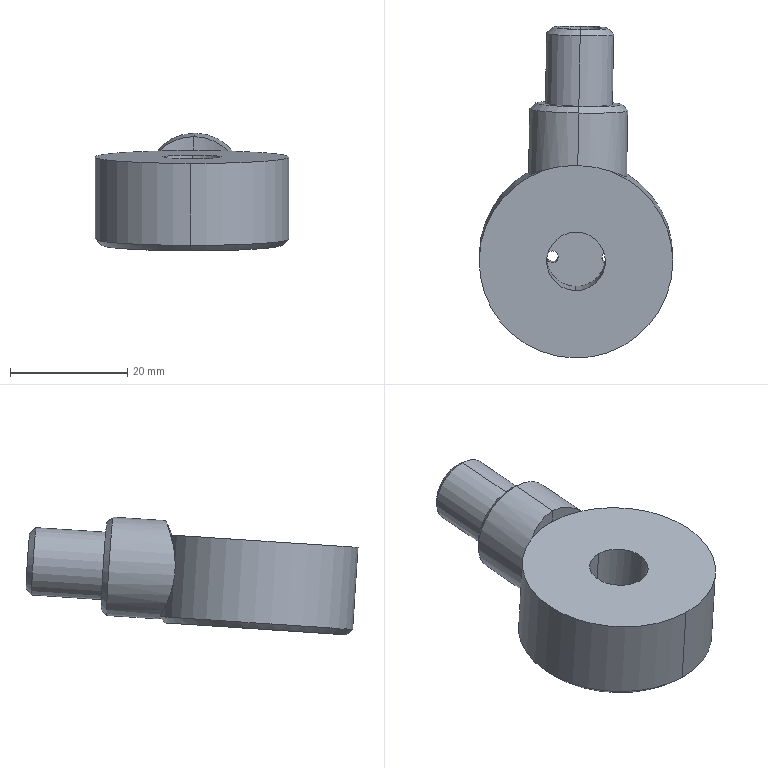Component | SolidWorks | LEDAlarm-1_RotatingHead-1 | 3 solids | 32 faces | box 33 x 56.59 x 20.06 mm | volume 13898 mm3 | cylinder 18 | plane 8 | cone 6 | commonest cylinder face diameters 11.5 x4 33 x4 2 x4 7.5 x2 16.8 x2 10 x2
build123d program:
from build123d import *

# Parameters (mm, degrees)
SKETCH1_R                = 16.5
SKETCH1_R_2              = 5
BOSS_EXTRUDE1_DEPTH      = 15
CHAMFER1_SIZE            = 1
EXTRUDE_THIN1_REACH      = 50.438
EXTRUDE_THIN1_END_RADIUS = 16.5
SKETCH3_R                = 8.4
SKETCH3_R_2              = 5.75
SKETCH4_R                = 5.75
SKETCH4_R_2              = 3.75
EXTRUDE_THIN2_DEPTH      = 13
CHAMFER2_SIZE            = 1
CHAMFER3_SIZE            = 1
BOSS_EXTRUDE2_START      = -4
SKETCH5_R                = 5
BOSS_EXTRUDE2_DEPTH      = 4
SKETCH6_R                = 1
CUT_EXTRUDE1_DEPTH       = 4


with BuildPart() as part:
    # Sketch1 → Boss-Extrude1 (new body)
    with BuildSketch(Plane.XY):
        Circle(SKETCH1_R)
        Circle(SKETCH1_R_2, mode=Mode.SUBTRACT)
    extrude(amount=BOSS_EXTRUDE1_DEPTH)

    # Chamfer1
    chamfer1_edges = [part.edges().sort_by_distance(p)[0] for p in [
        (-16.5, 0, 15),
    ]]
    chamfer(chamfer1_edges, length=CHAMFER1_SIZE)

    # Sketch5 → Boss-Extrude2 (add)
    with BuildSketch(Plane.XY.offset(15).offset(BOSS_EXTRUDE2_START)):
        Circle(SKETCH5_R)
    extrude(amount=BOSS_EXTRUDE2_DEPTH)

    # Sketch6 → Cut-Extrude1 (cut)
    with BuildSketch(Plane.XY.offset(15)):
        with Locations((0, -5.424)):
            Circle(SKETCH6_R)
        with Locations((0, 4.013)):
            Circle(SKETCH6_R)
    extrude(amount=-CUT_EXTRUDE1_DEPTH, mode=Mode.SUBTRACT)


with BuildPart() as body_2:
    # Extrude-Thin1: up to this cylinder (the profile starts outside it)
    extrude_thin1_end = Plane(origin=(0, 0, -2.162), z_dir=(0, 0, -1)) * Cylinder(EXTRUDE_THIN1_END_RADIUS, 134.876, mode=Mode.PRIVATE)
    # Sketch3 → Extrude-Thin1 (new, up to the surface)
    with BuildSketch(Plane.ZY.offset(26.5), mode=Mode.PRIVATE) as extrude_thin1_sk1:
        with Locations((6, 0)):
            Circle(SKETCH3_R)
        with Locations((6, 0)):
            Circle(SKETCH3_R_2, mode=Mode.SUBTRACT)
    extrude_thin1_tool1 = extrude(extrude_thin1_sk1.sketch, amount=-EXTRUDE_THIN1_REACH, mode=Mode.PRIVATE) - extrude_thin1_end
    add(extrude_thin1_tool1.solids().sort_by_distance((-26.5, 0, -2.162))[0])

    # Chamfer2
    chamfer2_edges = [body_2.edges().sort_by_distance(p)[0] for p in [
        (-26.5, 0, -2.4),
    ]]
    chamfer(chamfer2_edges, length=CHAMFER2_SIZE)


with BuildPart() as body_3:
    # Sketch4 → Extrude-Thin2 (new body)
    with BuildSketch(Plane.ZY.offset(26.5)):
        with Locations((6, 0)):
            Circle(SKETCH4_R)
        with Locations((6, 0)):
            Circle(SKETCH4_R_2, mode=Mode.SUBTRACT)
    extrude(amount=EXTRUDE_THIN2_DEPTH)

    # Chamfer3
    chamfer3_edges = [body_3.edges().sort_by_distance(p)[0] for p in [
        (-39.5, 0, 0.25),
    ]]
    chamfer(chamfer3_edges, length=CHAMFER3_SIZE)


solid = Compound([part.part, body_2.part, body_3.part])

# Placed as in the assembly
solid = solid.moved(Location((826.947, 455.702, 430.35), (-176.232, -0.005637, 91.056)))